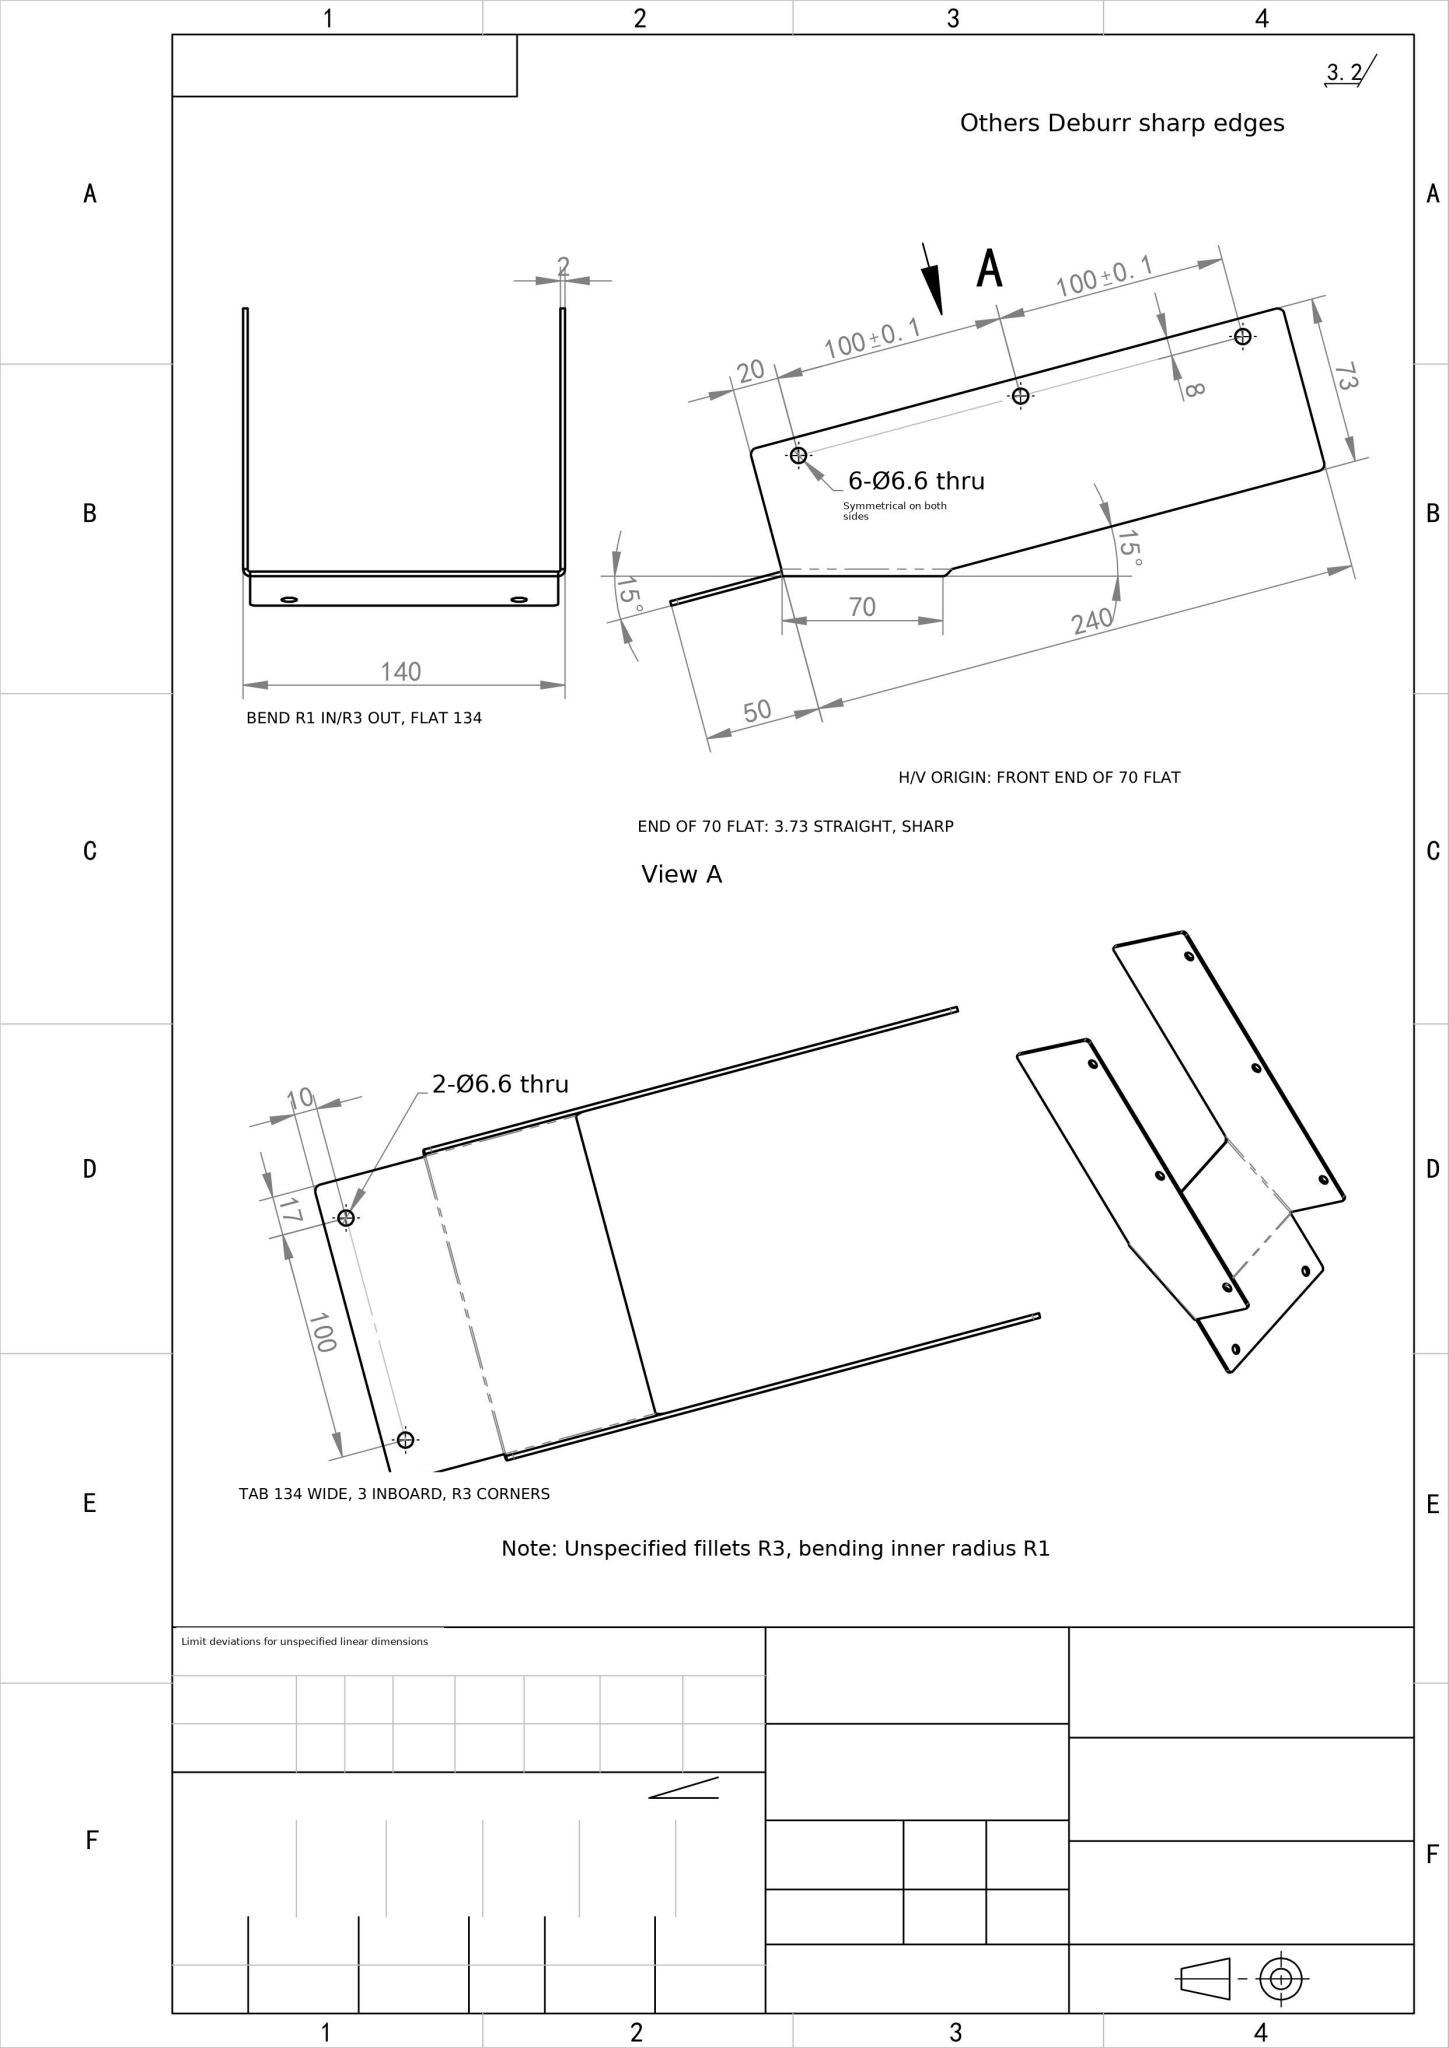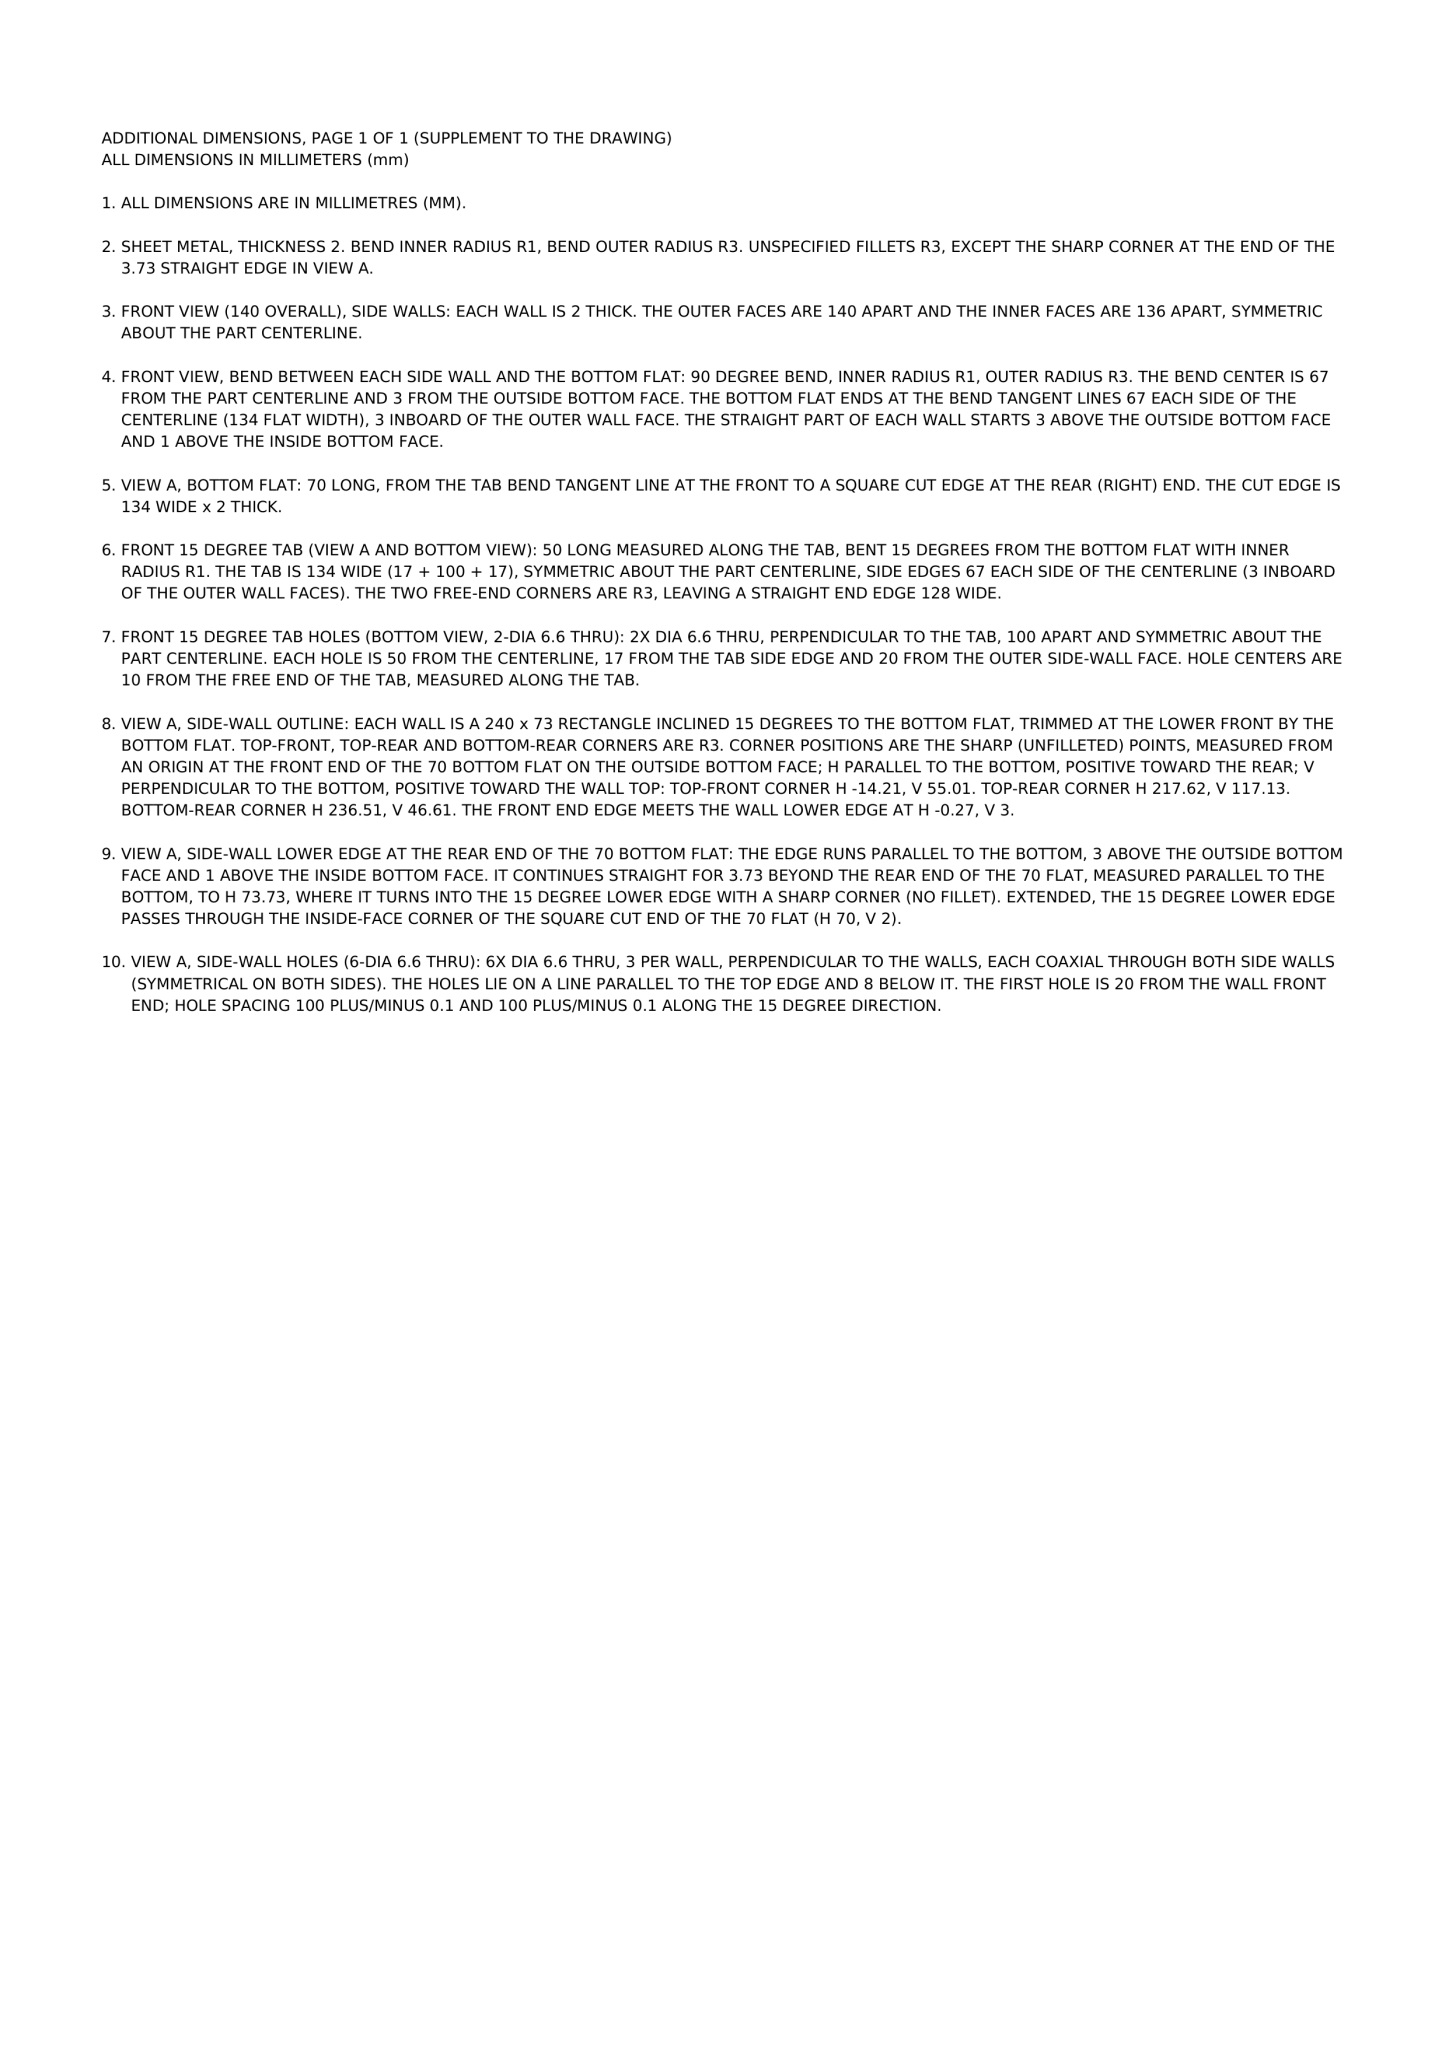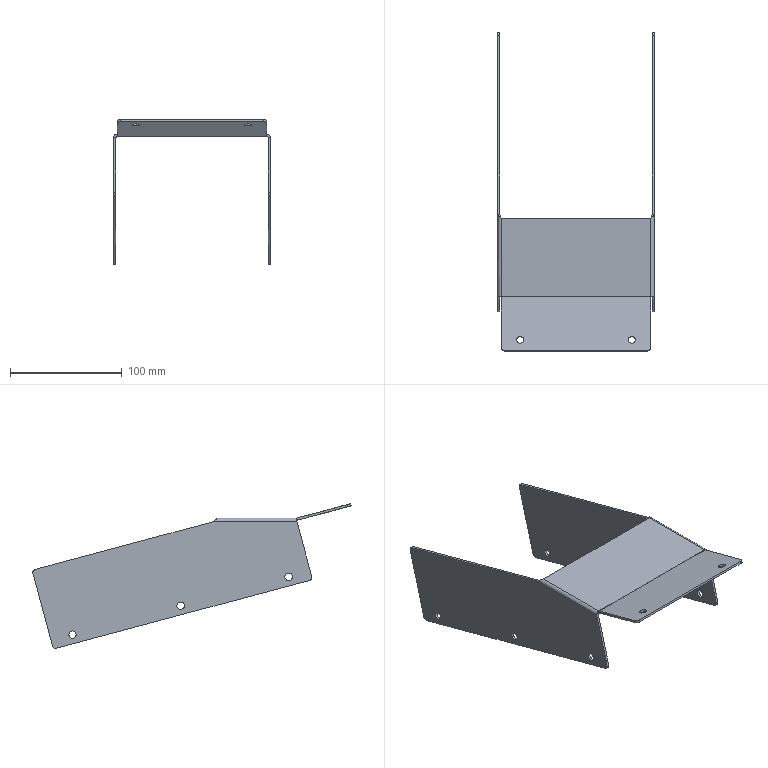Part | NX | mm | 1 solid | 57 faces | box 140 x 284.53 x 129.33 mm | volume 99863 mm3 | cylinder 31 | plane 22 | spline 4 | commonest cylinder face diameters 6.6 x16 6 x12 2 x3